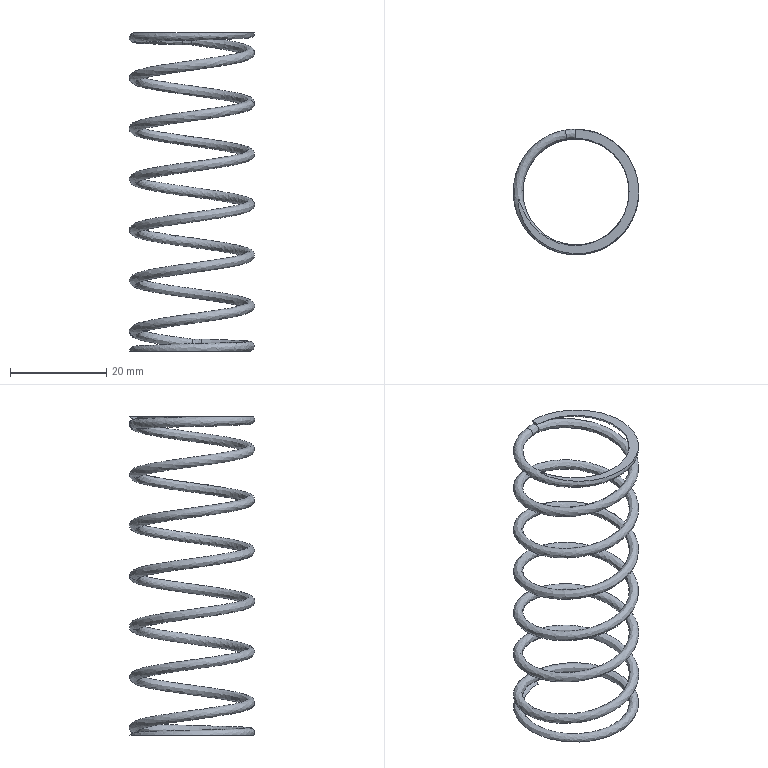Component | NX | SPRING | 1 solid | 9 faces | volume 1749 mm3 | spline 5 | plane 4